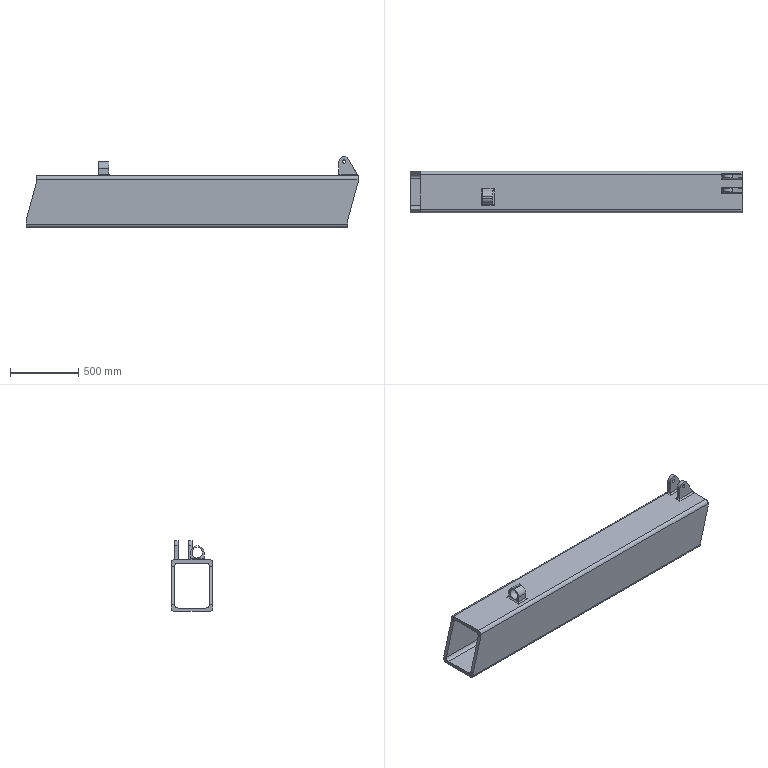Component | NX | ARM_SECTION_1 | 1 solid | 56 faces | volume 77251586 mm3 | plane 30 | cylinder 25 | spline 1 | commonest cylinder face diameters 20 x10 50 x8 76.2 x3 101.6 x2 25.4 x2